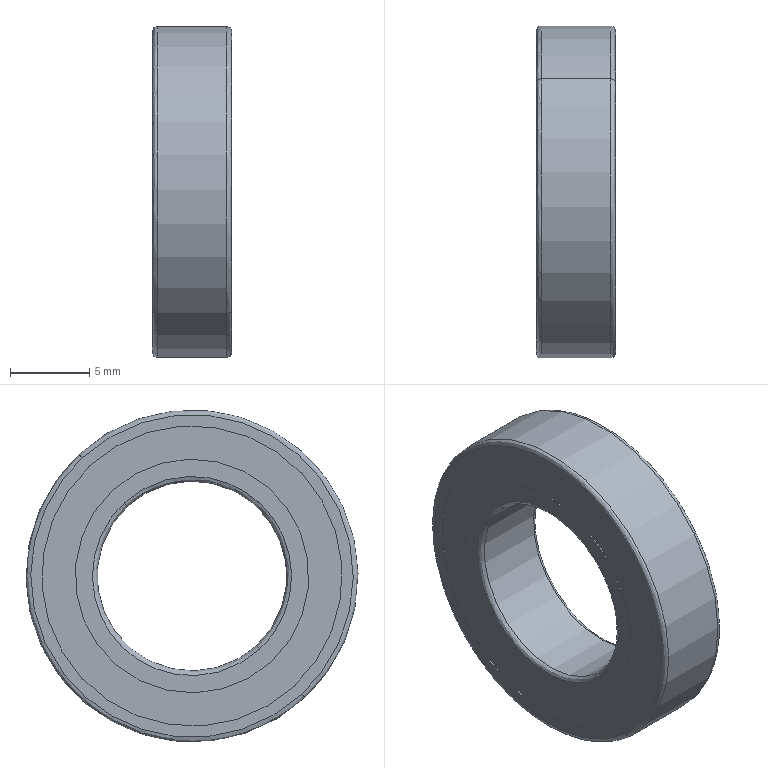Component | SolidWorks | DriveAxis-1_SB6801ZZ_2_14-1 | 1 solid | 26 faces | volume 1150 mm3 | cylinder 12 | spline 8 | plane 6 | commonest cylinder face diameters 19 x4 14.78 x4 21 x2 12 x2